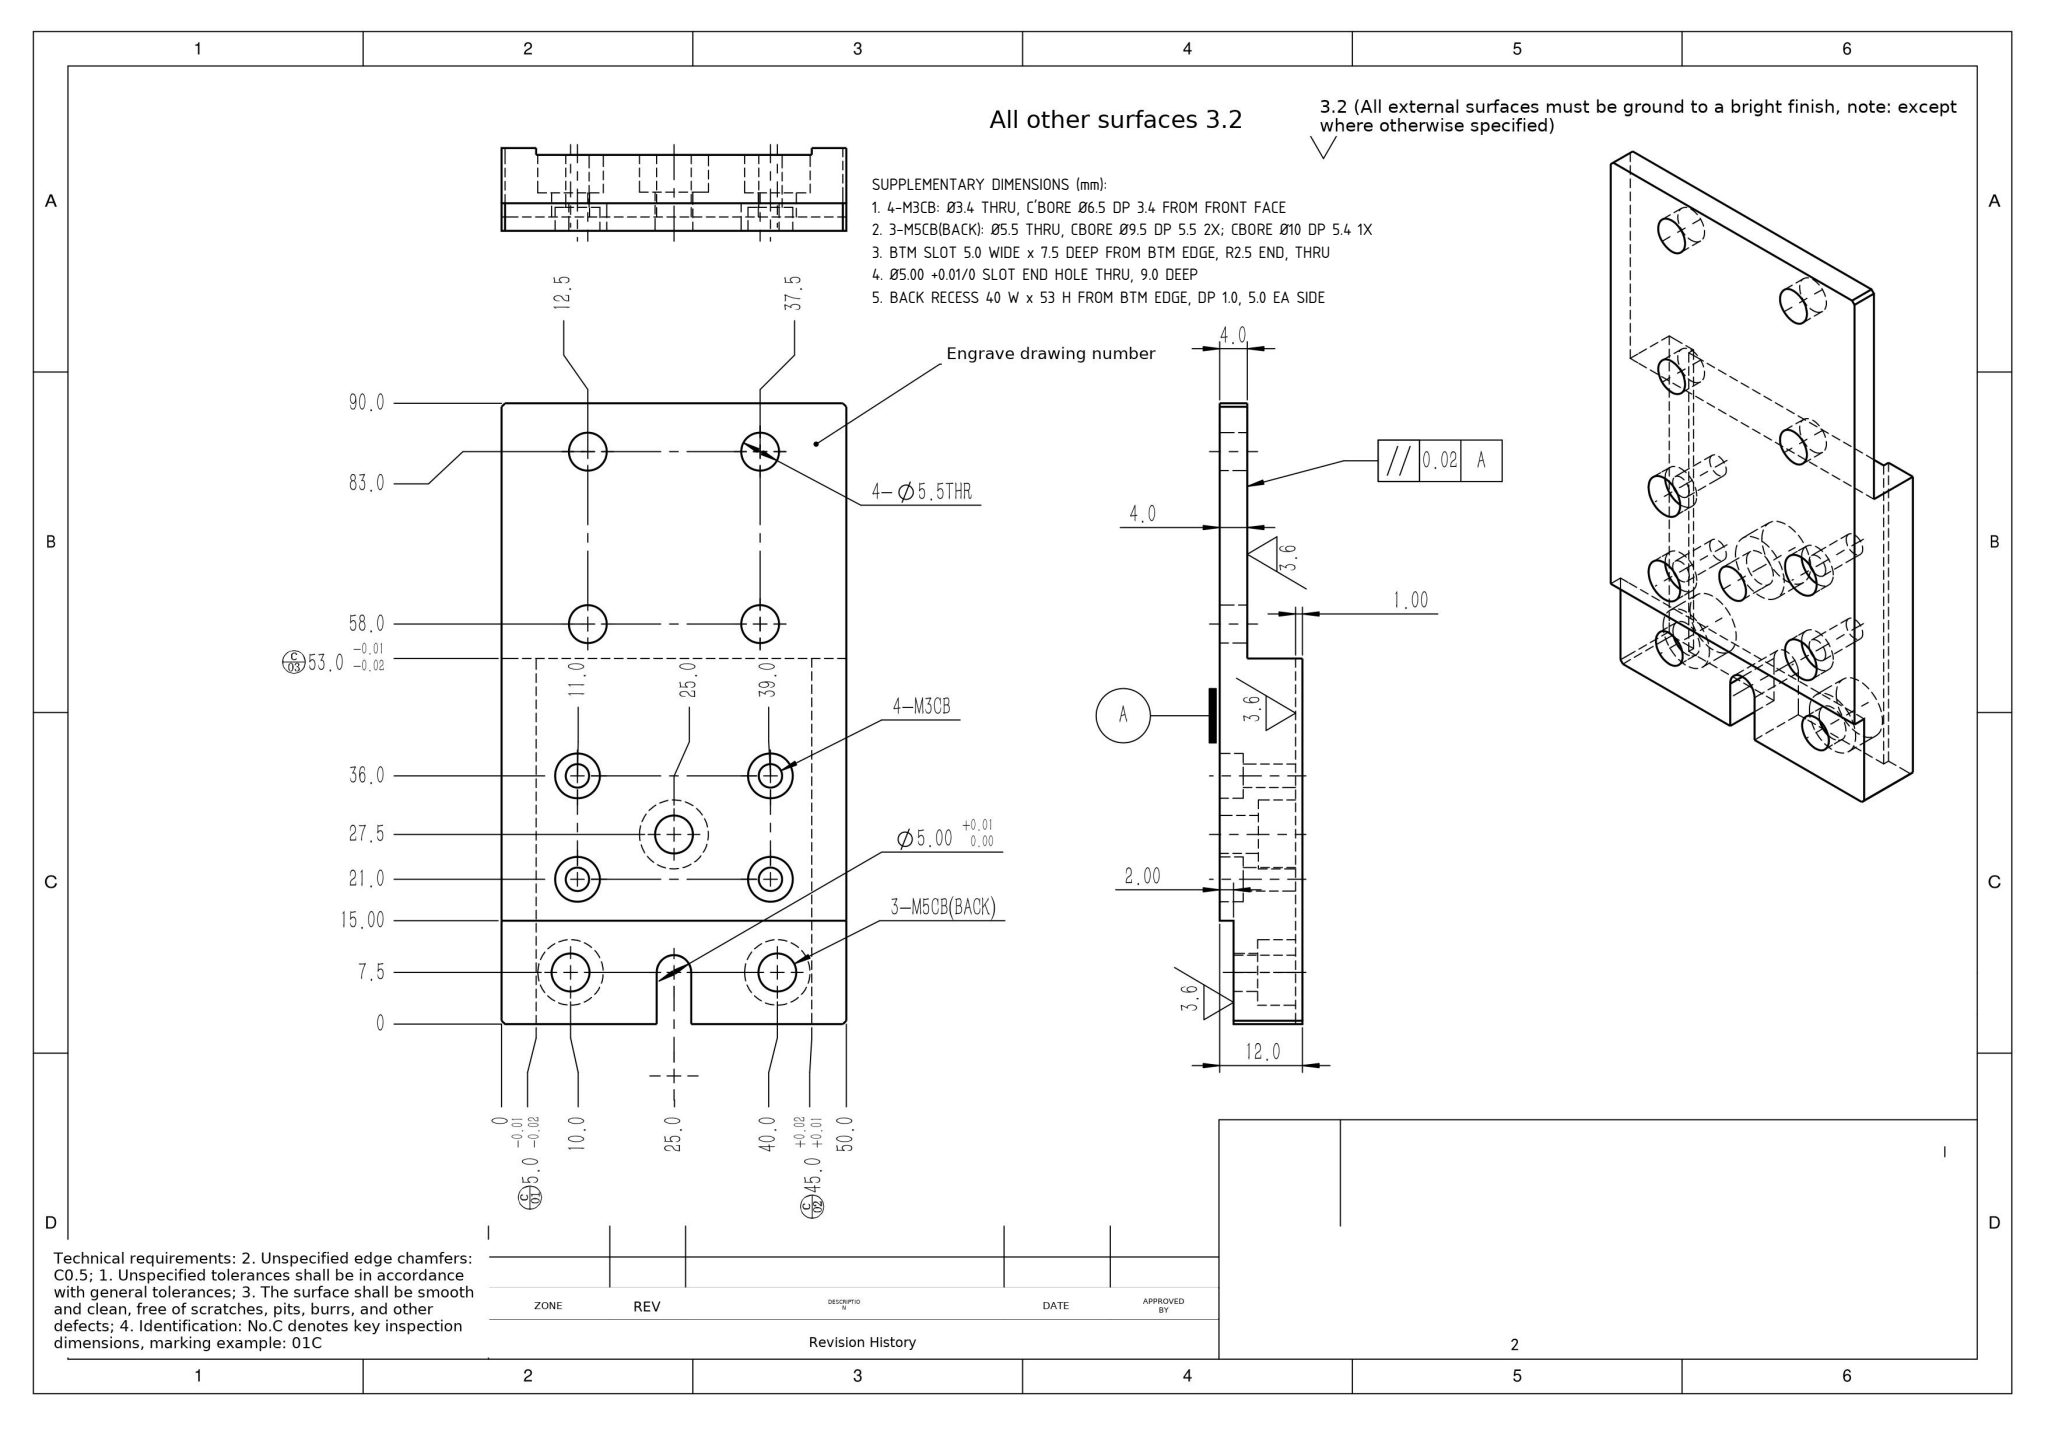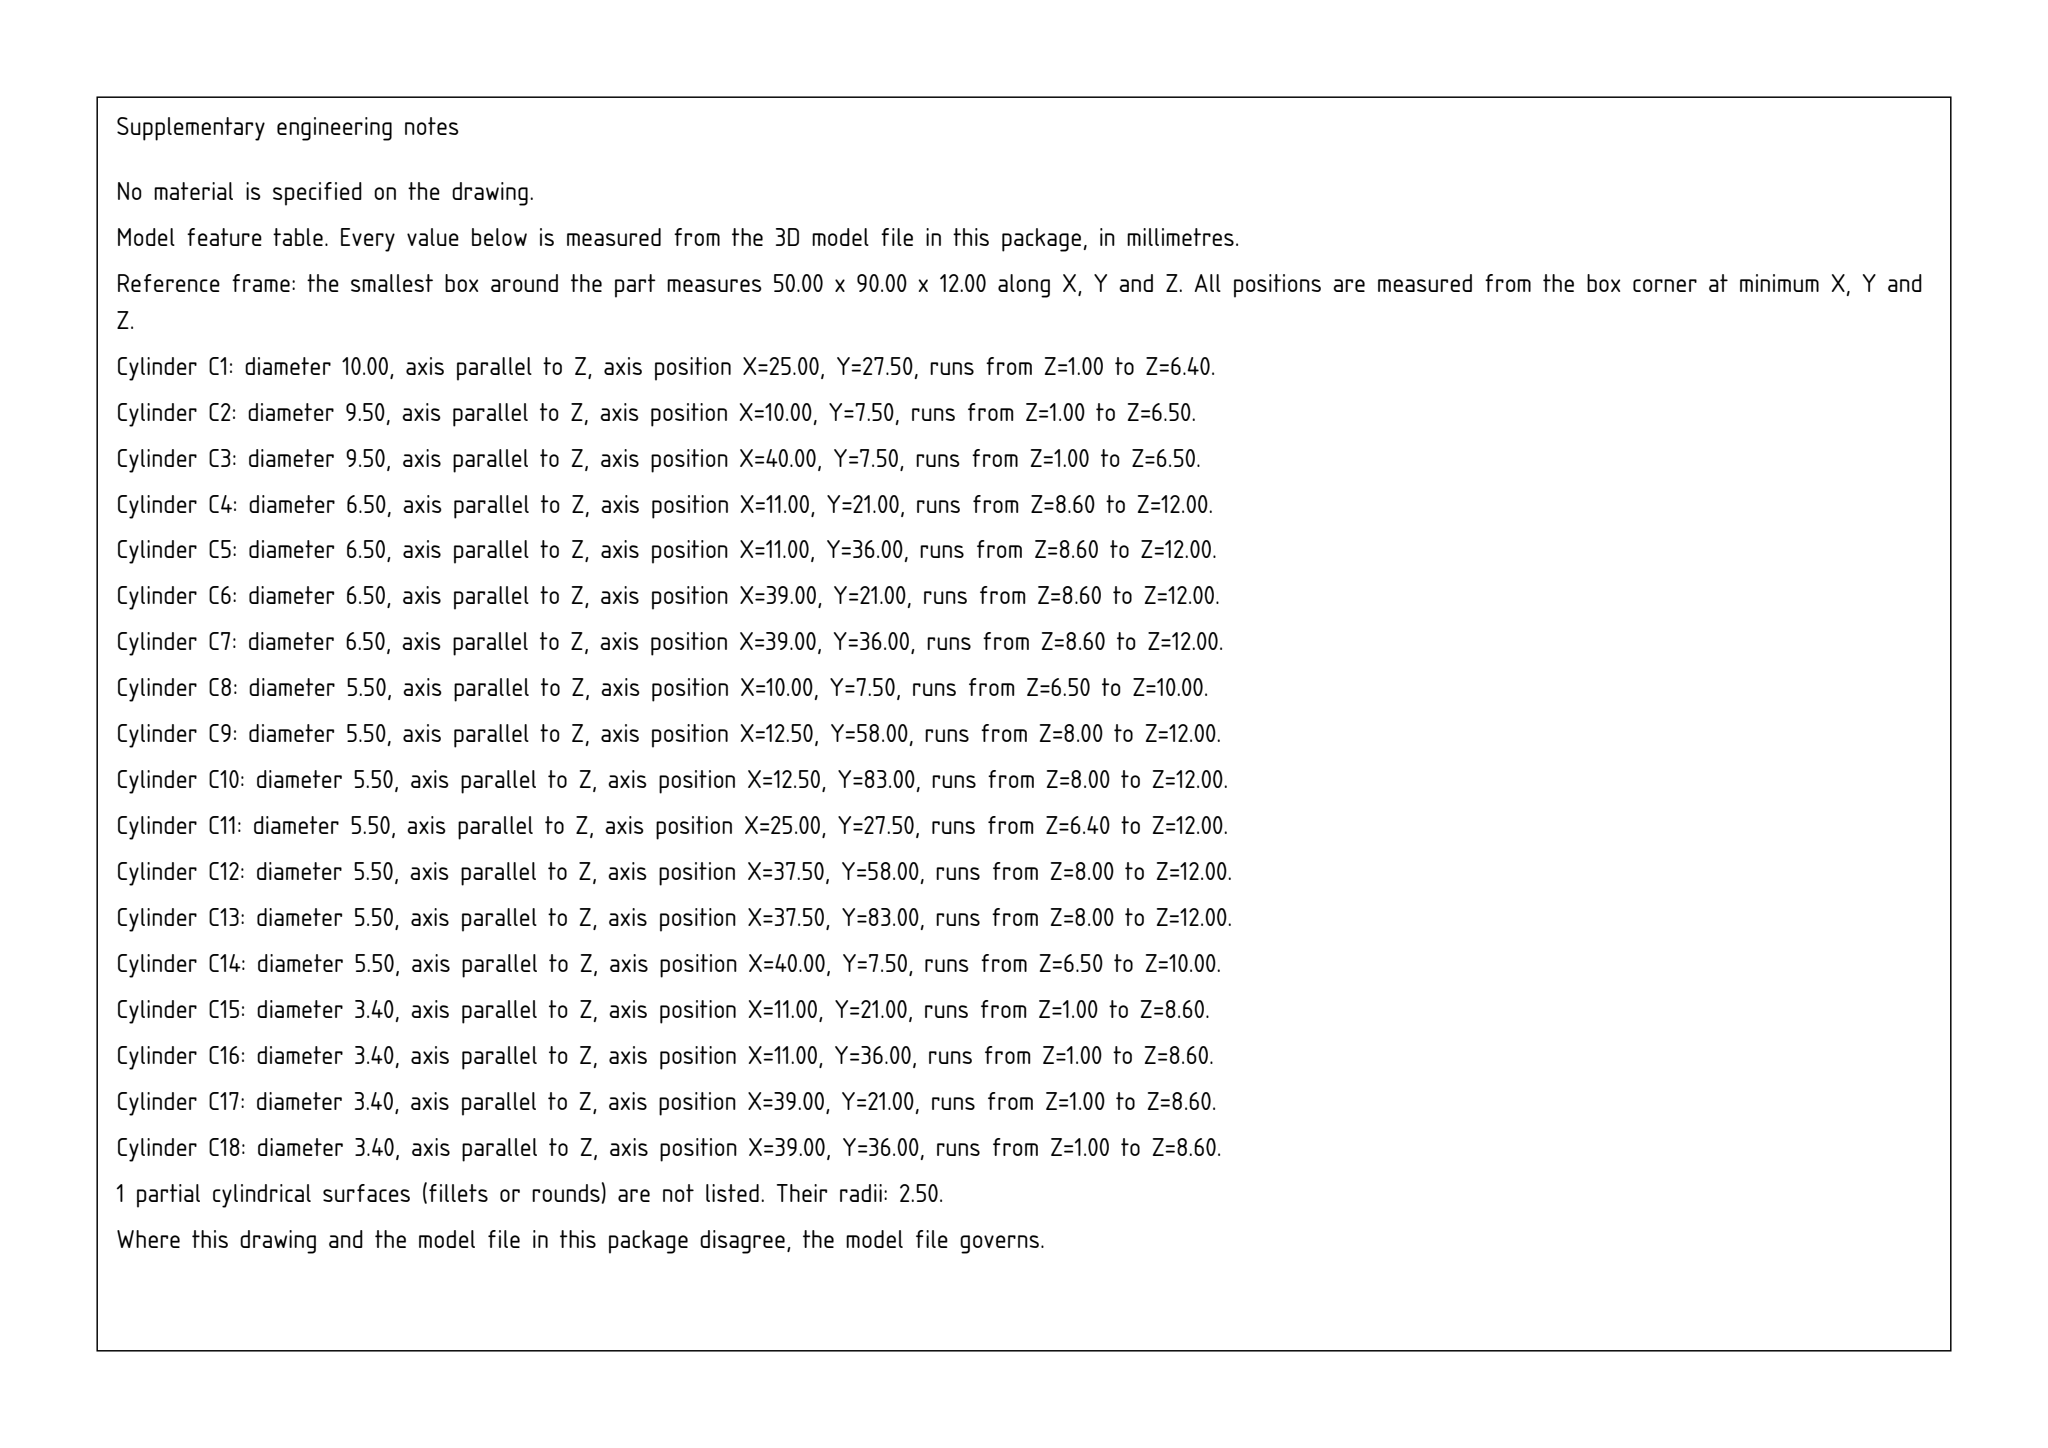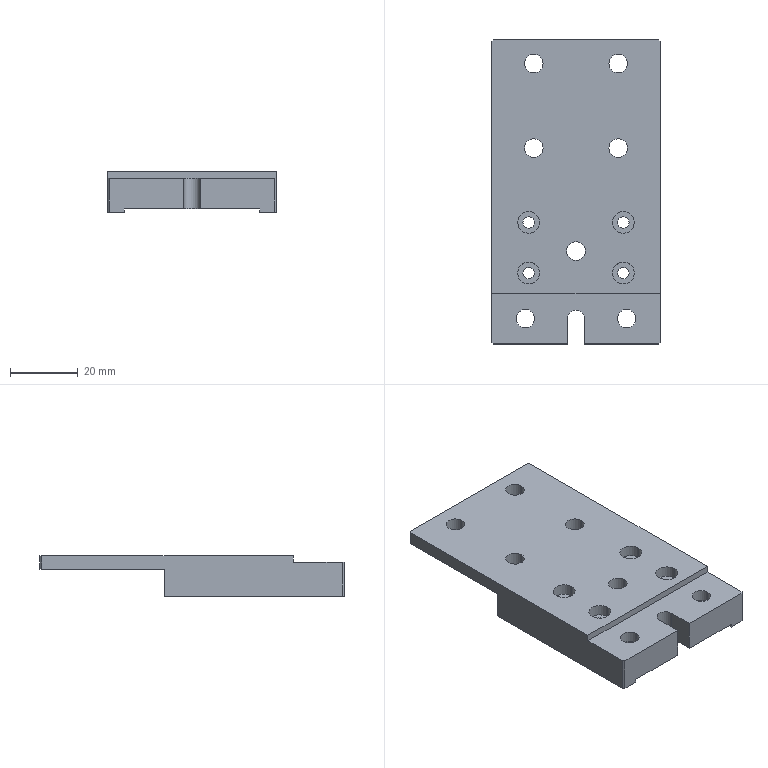Part | SolidWorks | mm | 1 solid | 65 faces | box 50 x 90 x 12 mm | volume 32540 mm3 | cylinder 37 | plane 28 | commonest cylinder face diameters 5.5 x14 3.4 x8 6.5 x8 9.5 x4 10 x2 5 x1
build123d program:
from build123d import *

# Parameters (mm, degrees)
SKETCH1_W                                           = 50
SKETCH1_H                                           = 60
BOSS_EXTRUDE1_DEPTH                                 = 12
SKETCH2_W                                           = 50
SKETCH2_H                                           = 15
CUT_EXTRUDE1_DEPTH                                  = 2
CYLINDRICAL_COUNTERSUNK_HOLE_FOR_M5_HEX_D           = 5.5
CYLINDRICAL_COUNTERSUNK_HOLE_FOR_M5_HEX_CBORE_D     = 9.5
CYLINDRICAL_COUNTERSUNK_HOLE_FOR_M5_HEX_CBORE_DEPTH = 6.5
LPATTERN1_COUNT                                     = 2
LPATTERN1_PITCH                                     = 30
SKETCH5_W                                           = 40
SKETCH5_H                                           = 60
CUT_EXTRUDE2_DEPTH                                  = 1
CUT_EXTRUDE3_DEPTH                                  = 79.74
M3_HEX_SOCKET_HEAD_CAP_SCREW_CBORE1_D               = 3.4
M3_HEX_SOCKET_HEAD_CAP_SCREW_CBORE1_CBORE_D         = 6.5
M3_HEX_SOCKET_HEAD_CAP_SCREW_CBORE1_CBORE_DEPTH     = 3.4
LPATTERN2_COUNT                                     = 2
LPATTERN2_PITCH                                     = 28
LPATTERN2_COUNT_DIR2                                = 2
LPATTERN2_PITCH_DIR2                                = 15
SKETCH9_W                                           = 15
SKETCH9_H                                           = 15
BOSS_EXTRUDE2_DEPTH                                 = 12
M5_HEX_SOCKET_HEAD_CAP_SCREW_CBORE1_D               = 5.5
M5_HEX_SOCKET_HEAD_CAP_SCREW_CBORE1_CBORE_D         = 10
M5_HEX_SOCKET_HEAD_CAP_SCREW_CBORE1_CBORE_DEPTH     = 5.4
SKETCH14_W                                          = 15
SKETCH14_H                                          = 15
CUT_EXTRUDE4_DEPTH                                  = 80.019
BOSS_EXTRUDE3_DEPTH                                 = 30
SKETCH16_W                                          = 8
SKETCH16_H                                          = 35
CUT_EXTRUDE5_DEPTH                                  = 104.653
F_5_5_5_5_DIAMETER_HOLE1_D                          = 5.5
F_5_5_5_5_DIAMETER_HOLE1_DEPTH                      = 15
F_5_5_5_5_DIAMETER_HOLE1_TIP                        = 1.652
SKETCH19_W                                          = 50
SKETCH19_H                                          = 8
CUT_EXTRUDE6_DEPTH                                  = 2
CHAMFER1_SIZE                                       = 0.5


with BuildPart() as part:
    # Sketch1 → Boss-Extrude1 (new body)
    with BuildSketch(Plane.XY):
        with Locations((25, 30)):
            Rectangle(SKETCH1_W, SKETCH1_H)
    extrude(amount=BOSS_EXTRUDE1_DEPTH)

    # Sketch2 → Cut-Extrude1 (cut)
    with BuildSketch(Plane.XY.offset(12)):
        with Locations((25, 7.5)):
            Rectangle(SKETCH2_W, SKETCH2_H)
    extrude(amount=-CUT_EXTRUDE1_DEPTH, mode=Mode.SUBTRACT)

    # Cylindrical countersunk hole for M5 Hex (through all)
    with Locations(Plane(origin=(0, 0, 0), x_dir=(-1, 0, 0), z_dir=(0, 0, -1))):
        with Locations((-10, 7.5)):
            cylindrical_countersunk_hole_for_m5_hex = CounterBoreHole(CYLINDRICAL_COUNTERSUNK_HOLE_FOR_M5_HEX_D / 2, CYLINDRICAL_COUNTERSUNK_HOLE_FOR_M5_HEX_CBORE_D / 2, CYLINDRICAL_COUNTERSUNK_HOLE_FOR_M5_HEX_CBORE_DEPTH)

    # LPattern1: Cylindrical countersunk hole for M5 Hex ×2
    with Locations(*[(i * LPATTERN1_PITCH, 0, 0) for i in range(1, LPATTERN1_COUNT)]):
        add(cylindrical_countersunk_hole_for_m5_hex, mode=Mode.SUBTRACT)

    # Sketch5 → Cut-Extrude2 (cut)
    with BuildSketch(Plane(origin=(0, 0, 0), x_dir=(-1, 0, 0), z_dir=(0, 0, -1))):
        with Locations((-25, 30)):
            Rectangle(SKETCH5_W, SKETCH5_H)
    extrude(amount=-CUT_EXTRUDE2_DEPTH, mode=Mode.SUBTRACT)

    # Sketch6 → Cut-Extrude3 (cut, through all)
    with BuildSketch(Plane.XY.offset(10)):
        with BuildLine():
            Line((22.5, -7.5), (22.5, 7.5))
            ThreePointArc((22.5, 7.5), (25, 10), (27.5, 7.5))
            Line((27.5, 7.5), (27.5, -7.5))
            ThreePointArc((27.5, -7.5), (25, -10), (22.5, -7.5))
        make_face()
    extrude(amount=-CUT_EXTRUDE3_DEPTH, mode=Mode.SUBTRACT)

    # M3 Hex Socket Head Cap Screw CBORE1 (through all)
    with Locations(Plane.XY.offset(12)):
        with Locations((39, 36)):
            m3_hex_socket_head_cap_screw_cbore1 = CounterBoreHole(M3_HEX_SOCKET_HEAD_CAP_SCREW_CBORE1_D / 2, M3_HEX_SOCKET_HEAD_CAP_SCREW_CBORE1_CBORE_D / 2, M3_HEX_SOCKET_HEAD_CAP_SCREW_CBORE1_CBORE_DEPTH)

    # LPattern2: M3 Hex Socket Head Cap Screw CBORE1 2 × 2
    with Locations(*[(-i * LPATTERN2_PITCH, -j * LPATTERN2_PITCH_DIR2, 0) for i in range(LPATTERN2_COUNT) for j in range(LPATTERN2_COUNT_DIR2) if (i, j) != (0, 0)]):
        add(m3_hex_socket_head_cap_screw_cbore1, mode=Mode.SUBTRACT)

    # Sketch9 → Boss-Extrude2 (add)
    with BuildSketch(Plane.XY.offset(12)):
        with Locations((-7.5, 52.5)):
            Rectangle(SKETCH9_W, SKETCH9_H)
    extrude(amount=-BOSS_EXTRUDE2_DEPTH)

    # M5 Hex Socket Head Cap Screw CBORE1 (through all)
    with Locations(Plane(origin=(0, 0, 1), x_dir=(-1, 0, 0), z_dir=(0, 0, -1))):
        with Locations((-25, 27.5)):
            CounterBoreHole(M5_HEX_SOCKET_HEAD_CAP_SCREW_CBORE1_D / 2, M5_HEX_SOCKET_HEAD_CAP_SCREW_CBORE1_CBORE_D / 2, M5_HEX_SOCKET_HEAD_CAP_SCREW_CBORE1_CBORE_DEPTH)

    # Sketch14 → Cut-Extrude4 (cut, through all)
    with BuildSketch(Plane.XY.offset(12)):
        with Locations((-7.5, 52.5)):
            Rectangle(SKETCH14_W, SKETCH14_H)
    extrude(amount=-CUT_EXTRUDE4_DEPTH, mode=Mode.SUBTRACT)

    # Sketch15 → Boss-Extrude3 (add)
    with BuildSketch(Plane(origin=(0, 60, 0), x_dir=(1, 0, 0), z_dir=(0, 1, 0))):
        Polygon((5, 0), (0, 0), (0, -12), (50, -12), (50, 0), (45, 0), (45, -1), (5, -1), align=None)
    extrude(amount=BOSS_EXTRUDE3_DEPTH)

    # Sketch16 → Cut-Extrude5 (cut, through all)
    with BuildSketch(Plane.ZY):
        with Locations((4, 70.5)):
            Rectangle(SKETCH16_W, SKETCH16_H)
    extrude(amount=-CUT_EXTRUDE5_DEPTH, mode=Mode.SUBTRACT)

    # 5.5 _5.5_ Diameter Hole1
    with Locations(Plane.XY.offset(12)):
        with Locations((37.5, 83), (12.5, 83), (37.5, 58), (12.5, 58)):
            Hole(F_5_5_5_5_DIAMETER_HOLE1_D / 2, depth=F_5_5_5_5_DIAMETER_HOLE1_DEPTH)
            with Locations((0, 0, -(F_5_5_5_5_DIAMETER_HOLE1_DEPTH + F_5_5_5_5_DIAMETER_HOLE1_TIP / 2))):  # 118° drill point
                Cone(0, F_5_5_5_5_DIAMETER_HOLE1_D / 2, F_5_5_5_5_DIAMETER_HOLE1_TIP, mode=Mode.SUBTRACT)

    # Sketch19 → Cut-Extrude6 (cut)
    with BuildSketch(Plane(origin=(0, 90, 0), x_dir=(1, 0, 0), z_dir=(0, 1, 0))):
        with Locations((25, -4)):
            Rectangle(SKETCH19_W, SKETCH19_H)
    extrude(amount=-CUT_EXTRUDE6_DEPTH, mode=Mode.SUBTRACT)

    # Chamfer1
    chamfer1_edges = [part.edges().sort_by_distance(p)[0] for p in [
        (0, 90, 10),
        (50, 90, 10),
        (50, 0, 5),
        (0, 0, 5),
    ]]
    chamfer(chamfer1_edges, length=CHAMFER1_SIZE)


solid = part.part